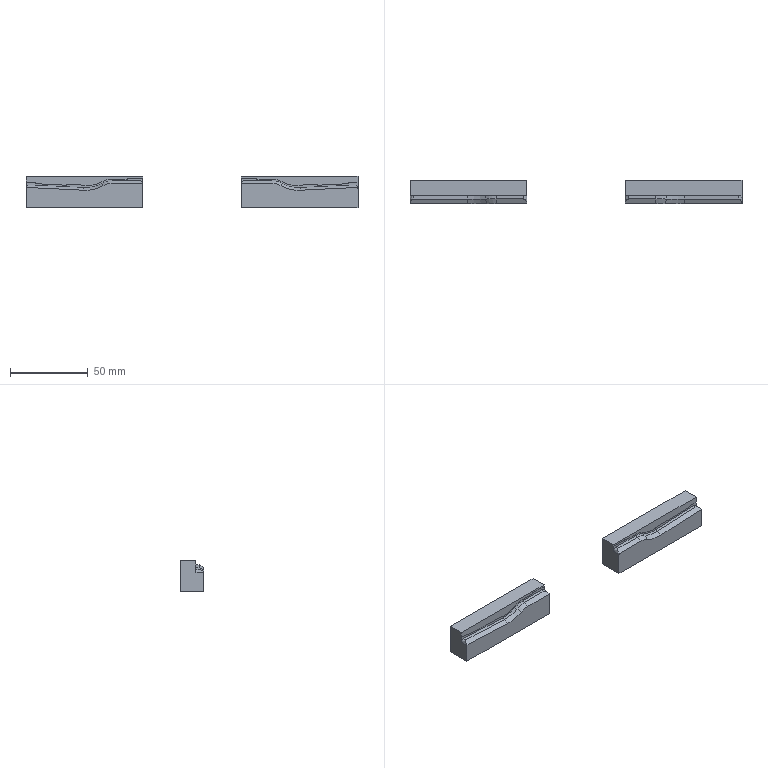Component | SolidWorks | Press-inFixture2-1 | 2 solids | 52 faces | volume 40274 mm3 | spline 20 | plane 16 | cylinder 8 | cone 8 | commonest cylinder face diameters 3.3 x8